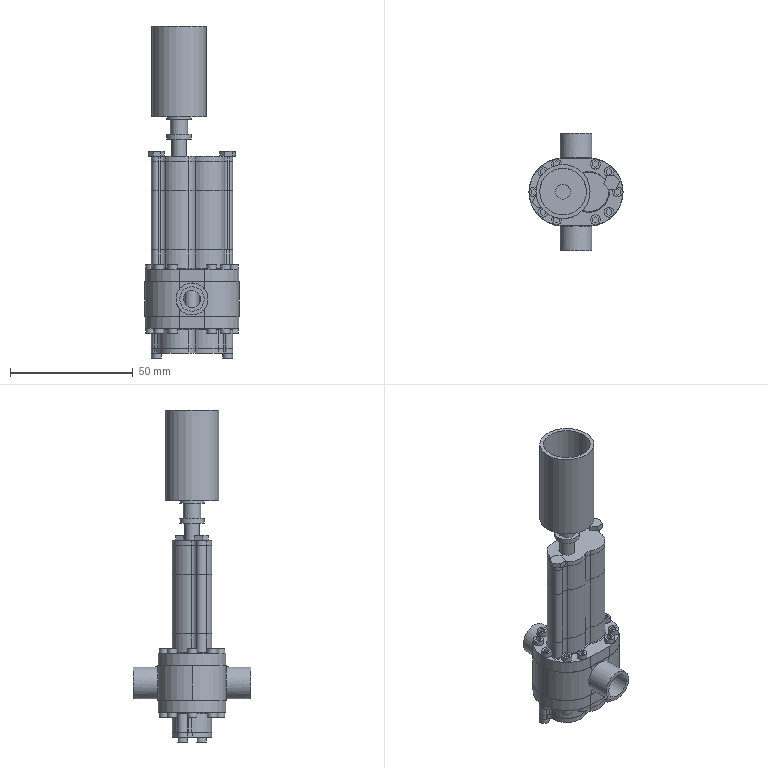Assembly | NX | mm | 40 component files | 58 solids | 939 faces | box 38.25 x 47.67 x 135 mm | volume 38643 mm3 | plane 354 | cylinder 305 | other 180 | cone 56 | torus 28 | sphere 16 | commonest cylinder face diameters 3 x56 4 x54 8.835 x36 16 x24 3.4 x20 6 x19 10 x12 5.568 x12
Bill of materials:
unnamed part 1 | 1 |  | Hollow obround/oval housing ring with a flat top flange face carrying 12 holes, an open central cavity with an internal step, and two hollow cylindrical tube stubs projecting from opposite sides on a common axis.
unnamed part 2 | 1 |  | Thin flat plate with a two-lobe (figure-eight) outline and two small ear tabs at diagonally opposite corners, each with a through hole. No central openings.
unnamed part 3 | 2 |  | Spur-gear-like toothed tube: a straight prism with external teeth all around and a large plain circular center bore. Its axial length is long compared with its diameter.
unnamed part 4 | 1 |  | Solid stepped round pin/shaft: a top cylindrical section, a slightly larger middle collar, a lower section near the top diameter, and a long thin small-diameter tip at the bottom.
unnamed part 5 | 1 |  | Cup-shaped hollow cylinder open at the top, with a closed bottom (it may have a rounded or chamfered outer edge) and a short, smaller coaxial stub underneath. The stub has a neck groove between two collars, and a central hole appears to pass through it.
unnamed part 6 | 2 |  | Resembles a ball bearing: concentric outer and inner rings with a set of spheres between them. No cage or shields are visible.
unnamed part 7 | 1 |  | Thin flat two-lobe (figure-eight) plate with diagonal ear tabs that have small through holes, plus one large circular through hole centered in one lobe.
unnamed part 8 | 1 |  | Thick block with a two-lobe (figure-eight) outline, two large parallel circular through bores centered in the lobes, and diagonal ear tabs with small through holes.
unnamed part 9 | 1 |  | Tall thin-walled shell with a two-lobe (figure-eight) outline, a single open two-lobe through cavity, and diagonal ear tabs with small through holes running the full height.
unnamed part 10 | 1 |  | Solid stepped round pin/shaft: a short top cylinder, a slightly larger collar section, a lower section near the top diameter, and a long thin reduced-diameter tip.
unnamed part 11 | 2 |  | Hex-head bolt-like part: a hexagonal head on a long, plain, round cylindrical shank with a slightly chamfered or rounded end.
unnamed part 12 | 1 |  | Obround flange plate with 12 through holes around the edge, a raised obround boss/recessed rim on top with two small through holes inside it, and a stepped lower body below. The lower body has lobed sections and a small cylindrical protrusion.
unnamed part 13 | 2 |  | Three-lobed prismatic block with a constant cross-section: three round lobes spaced evenly around a center, joined by concave arcs, with a small round through-hole at the center.
unnamed part 14 | 1 |  | Oval (obround) flange plate with a raised boss shaped like a figure-eight on top and a shorter, narrower step underneath. The boss has two large round through-bores side by side and two small holes on opposite corner lobes. Ten smaller holes run around the flange edge.
unnamed part 15 | 22 |  | Stepped round pin: a long plain cylinder with a short, larger collar or head at one end and a chamfered edge at the other end.
Mates:
1. fix | cavity 1 component
2. concentric | cavity 1 edge | end_cover 1 edge
3. parallel | end_cover 1 face | cavity 1 face
4. concentric | end_cover 1 edge | small_cover 1 arc
5. concentric | end_cover 1 edge | small_cover 1 arc
6. parallel | front_cover 1 face | cavity 1 face
7. concentric | front_cover 1 edge | housing 1 edge
8. concentric | front_cover 1 edge | housing 1 edge
9. concentric | housing 1 edge | gear_rotor_cover 1 arc
10. concentric | gear_rotor_cover 1 arc | housing 1 edge
11. concentric | drive_end_small_cover 1 arc | gear_rotor_cover 1 edge
12. concentric | drive_end_small_cover 1 arc | gear_rotor_cover 1 edge
13. concentric | driven_shaft 1 edge | drive_end_small_cover 1 edge
14. touch align | drive_shaft 1 face | drive_end_small_cover 1 face
15. distance | drive_shaft 1 face | driven_shaft 1 face
16. touch align | rotor 2 face | driven_shaft 1 face
17. distance | end_cover 1 face | rotor 2 face
18. touch align | rotor 1 face | drive_shaft 1 face
19. distance | end_cover 1 face | rotor 1 face
20. touch align | gear 2 face | drive_shaft 1 face
21. center | gear 2 face | gear 2 face | drive_shaft 1 face | drive_shaft 1 face
22. touch align | gear 1 face | driven_shaft 1 face
23. center | gear 1 face | gear 1 face | driven_shaft 1 face | driven_shaft 1 face
24. touch align | pump_flange_fitting 1 face | drive_shaft 1 face
25. distance | pump_flange_fitting 1 face | drive_end_small_cover 1 face
26. concentric | drive_end_small_cover 1 edge | long_screw_m3 2 arc
27. parallel | long_screw_m3 2 face | front_cover 1 face
28. concentric | drive_end_small_cover 1 edge | long_screw_m3 1 arc
29. parallel | long_screw_m3 1 face | front_cover 1 face
30. concentric | small_cover 1 edge | screw_m3x7 11 arc
31. concentric | small_cover 1 edge | screw_m3x7 10 arc
32. concentric | bearing 2 edge | end_cover 1 edge
33. concentric | end_cover 1 edge | bearing 1 edge